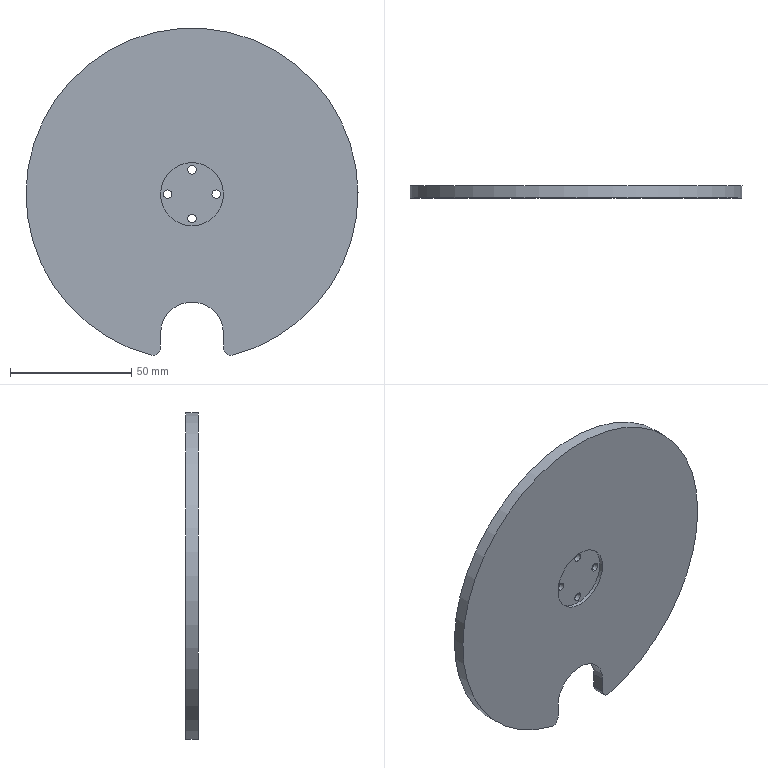CAM job | Mastercam | mm | 7 operations | part box 137 x 5 x 135.02
1. 2D High Speed (2D Area Mill) | 3 - 3 平铣刀
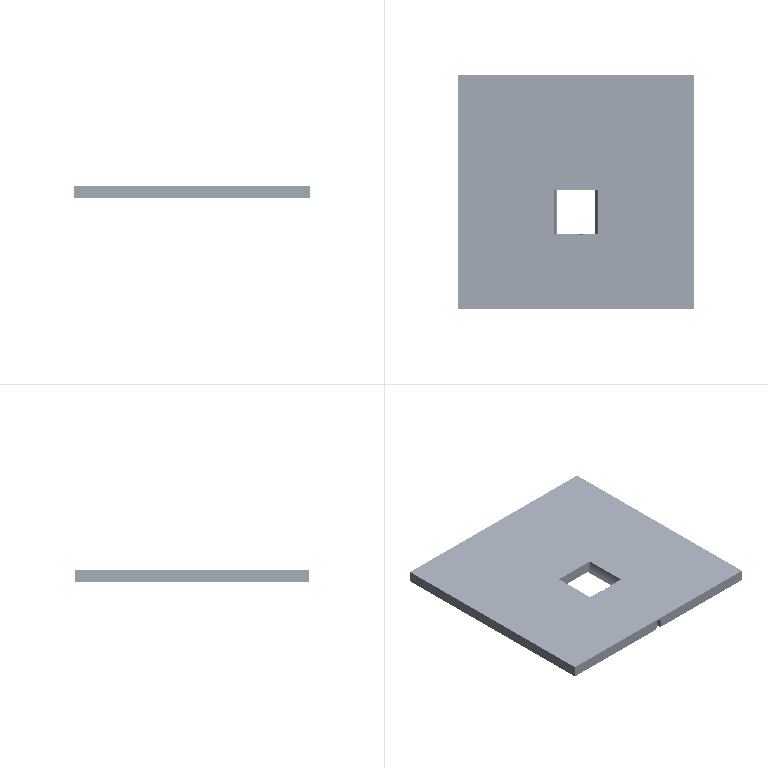2. 2D High Speed (2D Area Mill) | 3 - 3 平铣刀
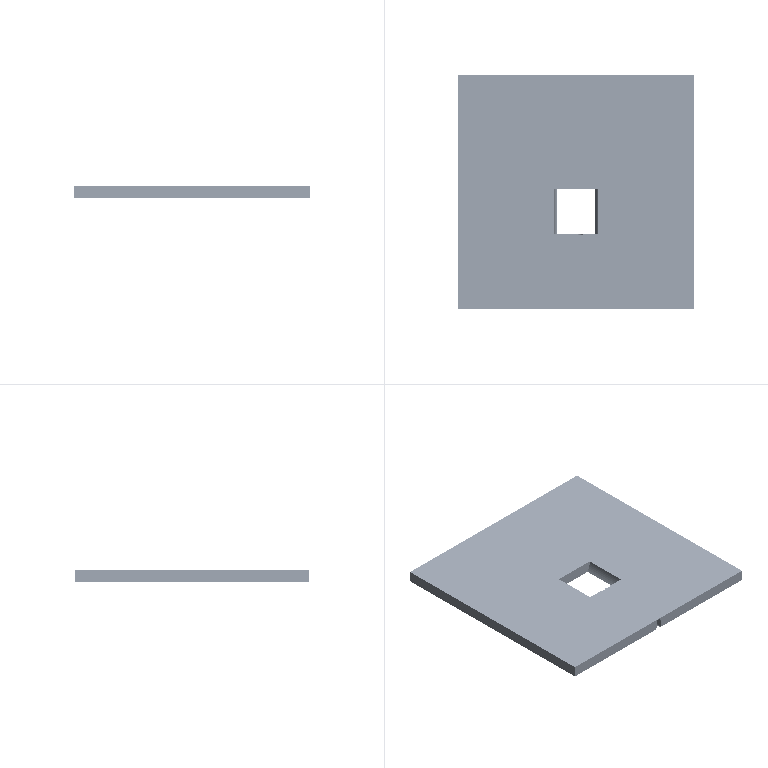3. Contour (2D) | 3 - 3 平铣刀
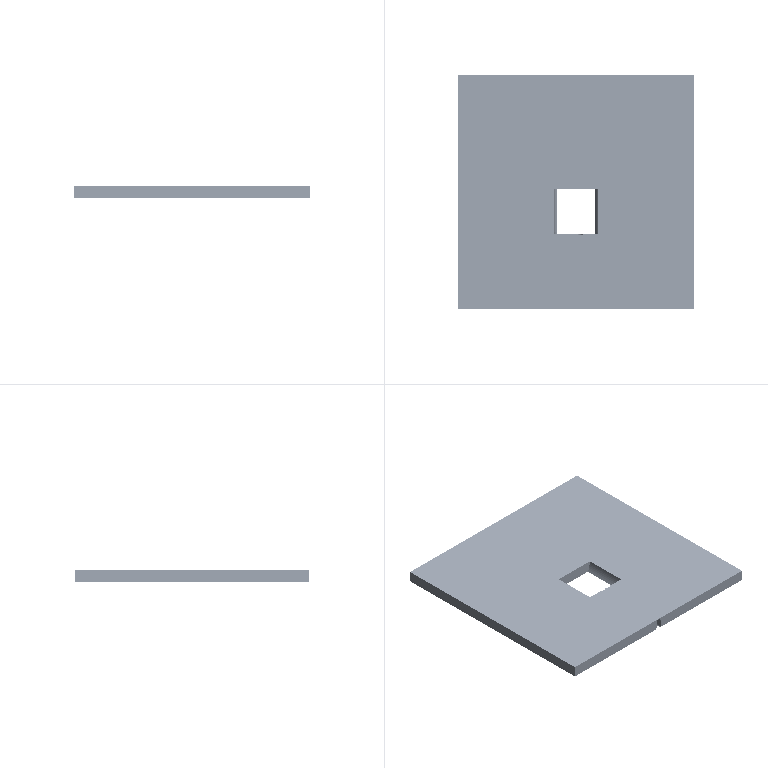4. Contour (Ramp) | 3 - 3 平铣刀
5. Contour (2D) | 3 - 3 平铣刀
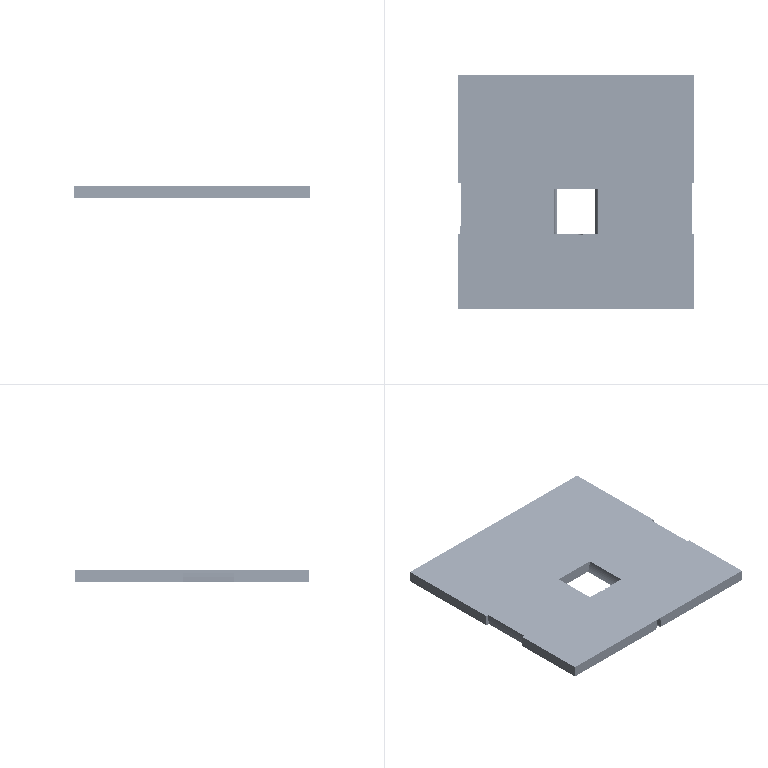6. Drill/Counterbore | 7 - 4 倒角刀
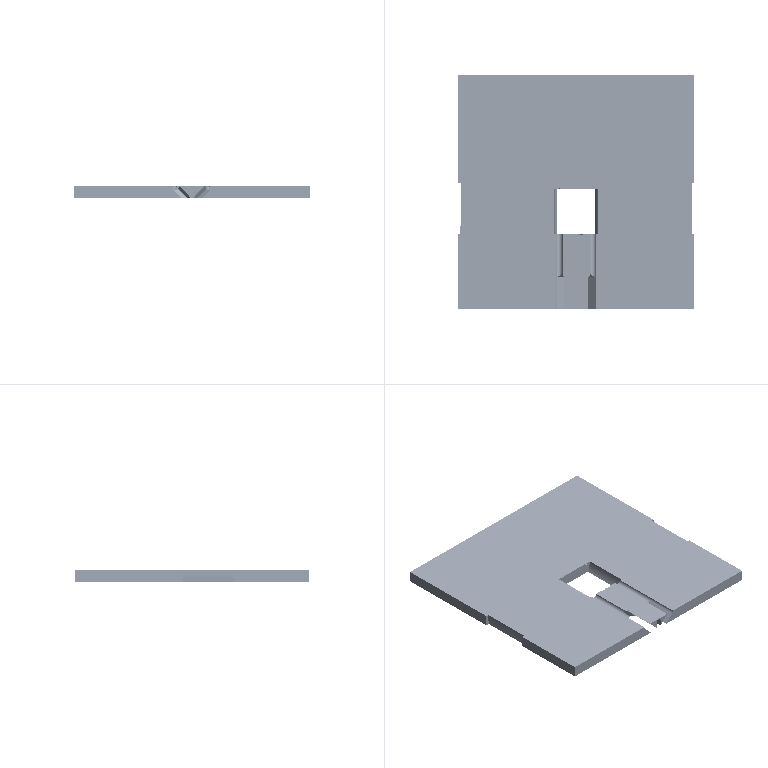7. Contour (2D chamfer) | 7 - 4 倒角刀